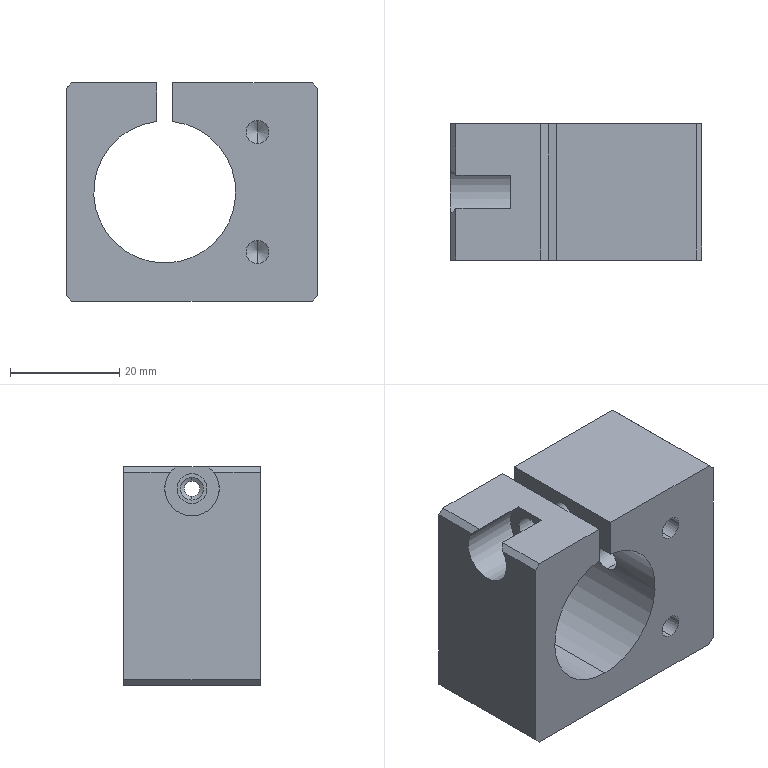Component | SolidWorks | MTCTV2104DJ006-000-0041ClampBlock-1 | 1 solid | 45 faces | box 46 x 25 x 40 mm | volume 29797 mm3 | cylinder 17 | plane 15 | cone 13 | commonest cylinder face diameters 4.2 x6 5 x6 5.5 x2 26 x2 10 x1
build123d program:
from build123d import *

# Parameters (mm, degrees)
SKETCH1_W                                           = 40
SKETCH1_H                                           = 25
BOSS_EXTRUDE1_DEPTH                                 = 46
M6_TAPPED_HOLE1_D                                   = 5
M6_TAPPED_HOLE1_DEPTH                               = 15
M6_TAPPED_HOLE1_TIP                                 = 1.502
SKETCH4_R                                           = 13
CUT_EXTRUDE1_DEPTH                                  = 57.045
SKETCH5_W                                           = 3
SKETCH5_H                                           = 20
CUT_EXTRUDE2_DEPTH                                  = 57.045
HOLE_SIZE_TYPE_OF_HEXAGON_SOCKET_HEAD_C_D           = 5.5
HOLE_SIZE_TYPE_OF_HEXAGON_SOCKET_HEAD_C_DEPTH       = 16.5
HOLE_SIZE_TYPE_OF_HEXAGON_SOCKET_HEAD_C_CBORE_D     = 10
HOLE_SIZE_TYPE_OF_HEXAGON_SOCKET_HEAD_C_CBORE_DEPTH = 11
M5_TAPPED_HOLE2_D                                   = 4.2
M5_TAPPED_HOLE2_DEPTH                               = 10.4
M5_TAPPED_HOLE2_TIP                                 = 1.262
M5_TAPPED_HOLE1_D                                   = 4.2
M5_TAPPED_HOLE1_DEPTH                               = 12.4
M5_TAPPED_HOLE1_TIP                                 = 1.262
CHAMFER1_SIZE                                       = 1
CHAMFER2_SIZE                                       = 1


with BuildPart() as part:
    # Sketch1 → Boss-Extrude1 (new body)
    with BuildSketch(Plane(origin=(0, 0, 0), x_dir=(0, 0, -1), z_dir=(1, 0, 0))):
        Rectangle(SKETCH1_W, SKETCH1_H)
    extrude(amount=BOSS_EXTRUDE1_DEPTH)

    # M6 Tapped Hole1
    with Locations(Plane.ZY):
        with Locations((-16, 0), (0, 0), (16, 0)):
            Hole(M6_TAPPED_HOLE1_D / 2, depth=M6_TAPPED_HOLE1_DEPTH)
            with Locations((0, 0, -(M6_TAPPED_HOLE1_DEPTH + M6_TAPPED_HOLE1_TIP / 2))):  # 118° drill point
                Cone(0, M6_TAPPED_HOLE1_D / 2, M6_TAPPED_HOLE1_TIP, mode=Mode.SUBTRACT)

    # Sketch4 → Cut-Extrude1 (cut, through all)
    with BuildSketch(Plane(origin=(0, 12.5, 0), x_dir=(1, 0, 0), z_dir=(0, 1, 0))):
        with Locations(Location((28, 0, 0), (0, 0, 270))):
            Circle(SKETCH4_R)
    extrude(amount=-CUT_EXTRUDE1_DEPTH, mode=Mode.SUBTRACT)

    # Sketch5 → Cut-Extrude2 (cut, through all)
    with BuildSketch(Plane(origin=(0, 12.5, 0), x_dir=(1, 0, 0), z_dir=(0, 1, 0))):
        with Locations((28, 10)):
            Rectangle(SKETCH5_W, SKETCH5_H)
    extrude(amount=-CUT_EXTRUDE2_DEPTH, mode=Mode.SUBTRACT)

    # Hole Size _Type of Hexagon Socket Head C
    with Locations(Plane(origin=(46, 0, 0), x_dir=(0, 0, -1), z_dir=(1, 0, 0))):
        with Locations((16, 0)):
            CounterBoreHole(HOLE_SIZE_TYPE_OF_HEXAGON_SOCKET_HEAD_C_D / 2, HOLE_SIZE_TYPE_OF_HEXAGON_SOCKET_HEAD_C_CBORE_D / 2, HOLE_SIZE_TYPE_OF_HEXAGON_SOCKET_HEAD_C_CBORE_DEPTH, depth=HOLE_SIZE_TYPE_OF_HEXAGON_SOCKET_HEAD_C_DEPTH)

    # M5 Tapped Hole2
    with Locations(Plane(origin=(26.5, 0, 0), x_dir=(0, 0, -1), z_dir=(1, 0, 0))):
        with Locations((16, 0)):
            Hole(M5_TAPPED_HOLE2_D / 2, depth=M5_TAPPED_HOLE2_DEPTH)
            with Locations((0, 0, -(M5_TAPPED_HOLE2_DEPTH + M5_TAPPED_HOLE2_TIP / 2))):  # 118° drill point
                Cone(0, M5_TAPPED_HOLE2_D / 2, M5_TAPPED_HOLE2_TIP, mode=Mode.SUBTRACT)

    # M5 Tapped Hole1
    with Locations(Plane(origin=(0, -12.5, 0), x_dir=(-1, 0, 0), z_dir=(0, -1, 0))):
        with Locations((-11, -11), (-11, 11)):
            Hole(M5_TAPPED_HOLE1_D / 2, depth=M5_TAPPED_HOLE1_DEPTH)
            with Locations((0, 0, -(M5_TAPPED_HOLE1_DEPTH + M5_TAPPED_HOLE1_TIP / 2))):  # 118° drill point
                Cone(0, M5_TAPPED_HOLE1_D / 2, M5_TAPPED_HOLE1_TIP, mode=Mode.SUBTRACT)

    # Chamfer1
    chamfer1_edges = [part.edges().sort_by_distance(p)[0] for p in [
        (46, 0, 20),
        (0, 0, 20),
        (0, 0, -20),
    ]]
    chamfer(chamfer1_edges, length=CHAMFER1_SIZE)

    # Chamfer2
    chamfer2_edges = [part.edges().sort_by_distance(p)[0] for p in [
        (46, -7.75, -20),
        (46, 7.75, -20),
    ]]
    chamfer(chamfer2_edges, length=CHAMFER2_SIZE)


solid = part.part

# Placed as in the assembly
solid = solid.moved(Location((31.798, -88.178, 265.447), (-180, 0, 180)))